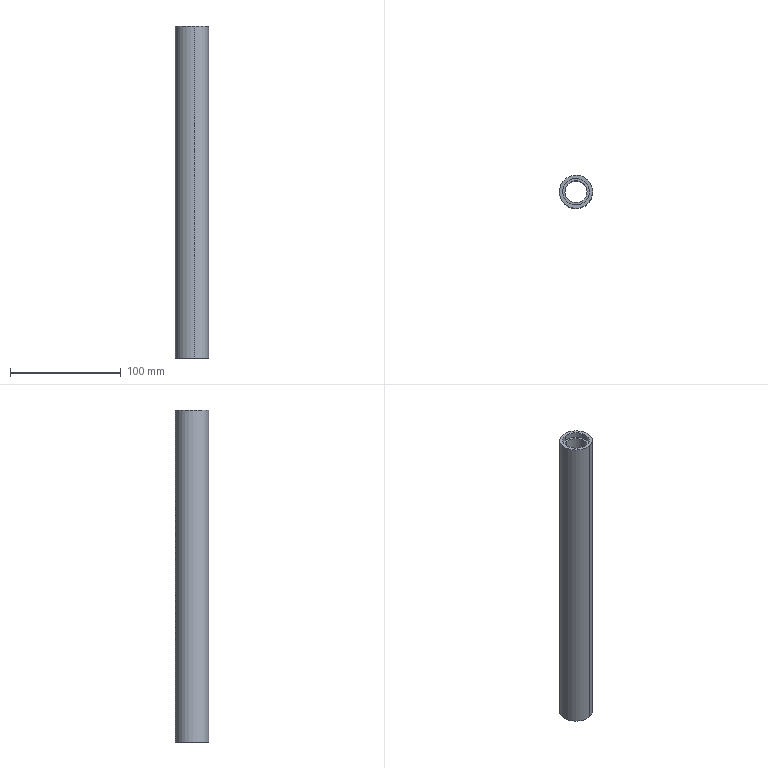Component | SolidWorks | KSD171005A-01-01-25-2 | 1 solid | 12 faces | box 30 x 30 x 300 mm | volume 116427 mm3 | cylinder 8 | plane 4 | commonest cylinder face diameters 24 x4 20 x2 30 x2 | material Aluminum
build123d program:
from build123d import *


with BuildPart() as part:
    # Sketch1 → Revolve1 (revolve)
    with BuildSketch(Plane.XY, mode=Mode.PRIVATE) as revolve1_sk:
        Polygon((0, 12), (0, 15), (300, 15), (300, 12), (295, 12), (295, 10), (5, 10), (5, 12), align=None)
    revolve(revolve1_sk.sketch.rotate(Axis((-43.14, 0, 0), (1, 0, 0)), 90), axis=Axis((-43.14, 0, 0), (1, 0, 0)))


solid = part.part

# Placed as in the assembly
solid = solid.moved(Location((-7.111, -139.27, 933), (0, 90, 0)))
STEP:
#1=CARTESIAN_POINT('',(-0.3647,-5.018,25.118));
#2=VERTEX_POINT('',#1);
#3=CARTESIAN_POINT('',(-0.1952,-5.948,25.118));
#4=VERTEX_POINT('',#3);
#5=CARTESIAN_POINT('',(-0.28,-5.483,25.118));
#6=DIRECTION('',(0.,-0.,-1.));
#7=DIRECTION('',(0.1794,-0.9838,0.));
#8=AXIS2_PLACEMENT_3D('',#5,#6,#7);
#9=CIRCLE('',#8,0.4724);
#10=EDGE_CURVE('',#2,#4,#9,.T.);
#11=ORIENTED_EDGE('',*,*,#10,.F.);
#12=CARTESIAN_POINT('',(-0.3647,-5.018,24.921));
#13=VERTEX_POINT('',#12);
#14=CARTESIAN_POINT('',(-0.3647,-5.018,23.223));
#15=DIRECTION('',(0.,-0.,-1.));
#16=VECTOR('',#15,39.37);
#17=LINE('',#14,#16);
#18=EDGE_CURVE('',#2,#13,#17,.T.);
#19=ORIENTED_EDGE('',*,*,#18,.T.);
#20=CARTESIAN_POINT('',(-0.1952,-5.948,24.921));
#21=VERTEX_POINT('',#20);
#22=CARTESIAN_POINT('',(-0.28,-5.483,24.921));
#23=DIRECTION('',(0.,-0.,-1.));
#24=DIRECTION('',(0.1794,-0.9838,0.));
#25=AXIS2_PLACEMENT_3D('',#22,#23,#24);
#26=CIRCLE('',#25,0.4724);
#27=EDGE_CURVE('',#13,#21,#26,.T.);
#28=ORIENTED_EDGE('',*,*,#27,.T.);
#29=CARTESIAN_POINT('',(-0.1952,-5.948,23.223));
#30=DIRECTION('',(0.,-0.,-1.));
#31=VECTOR('',#30,39.37);
#32=LINE('',#29,#31);
#33=EDGE_CURVE('',#4,#21,#32,.T.);
#34=ORIENTED_EDGE('',*,*,#33,.F.);
#35=EDGE_LOOP('',(#11,#19,#28,#34));
#36=FACE_OUTER_BOUND('',#35,.T.);
#37=CARTESIAN_POINT('',(-0.28,-5.483,23.223));
#38=DIRECTION('',(0.,-0.,-1.));
#39=DIRECTION('',(0.1794,-0.9838,0.));
#40=AXIS2_PLACEMENT_3D('',#37,#38,#39);
#41=CYLINDRICAL_SURFACE('',#40,0.4724);
#42=ADVANCED_FACE('',(#36),#41,.F.);
#43=CARTESIAN_POINT('',(-0.3506,-5.096,36.535));
#44=VERTEX_POINT('',#43);
#45=CARTESIAN_POINT('',(-0.2093,-5.87,36.535));
#46=VERTEX_POINT('',#45);
#47=CARTESIAN_POINT('',(-0.28,-5.483,36.535));
#48=DIRECTION('',(0.,-0.,-1.));
#49=DIRECTION('',(0.1794,-0.9838,0.));
#50=AXIS2_PLACEMENT_3D('',#47,#48,#49);
#51=CIRCLE('',#50,0.3937);
#52=EDGE_CURVE('',#44,#46,#51,.T.);
#53=ORIENTED_EDGE('',*,*,#52,.F.);
#54=CARTESIAN_POINT('',(-0.3506,-5.096,25.118));
#55=VERTEX_POINT('',#54);
#56=CARTESIAN_POINT('',(-0.3506,-5.096,23.223));
#57=DIRECTION('',(0.,-0.,-1.));
#58=VECTOR('',#57,39.37);
#59=LINE('',#56,#58);
#60=EDGE_CURVE('',#44,#55,#59,.T.);
#61=ORIENTED_EDGE('',*,*,#60,.T.);
#62=CARTESIAN_POINT('',(-0.2093,-5.87,25.118));
#63=VERTEX_POINT('',#62);
#64=CARTESIAN_POINT('',(-0.28,-5.483,25.118));
#65=DIRECTION('',(0.,-0.,-1.));
#66=DIRECTION('',(0.1794,-0.9838,0.));
#67=AXIS2_PLACEMENT_3D('',#64,#65,#66);
#68=CIRCLE('',#67,0.3937);
#69=EDGE_CURVE('',#55,#63,#68,.T.);
#70=ORIENTED_EDGE('',*,*,#69,.T.);
#71=CARTESIAN_POINT('',(-0.2093,-5.87,23.223));
#72=DIRECTION('',(0.,-0.,-1.));
#73=VECTOR('',#72,39.37);
#74=LINE('',#71,#73);
#75=EDGE_CURVE('',#46,#63,#74,.T.);
#76=ORIENTED_EDGE('',*,*,#75,.F.);
#77=EDGE_LOOP('',(#53,#61,#70,#76));
#78=FACE_OUTER_BOUND('',#77,.T.);
#79=CARTESIAN_POINT('',(-0.28,-5.483,23.223));
#80=DIRECTION('',(0.,-0.,-1.));
#81=DIRECTION('',(0.1794,-0.9838,0.));
#82=AXIS2_PLACEMENT_3D('',#79,#80,#81);
#83=CYLINDRICAL_SURFACE('',#82,0.3937);
#84=ADVANCED_FACE('',(#78),#83,.F.);
#85=CARTESIAN_POINT('',(-0.3647,-5.018,36.732));
#86=VERTEX_POINT('',#85);
#87=CARTESIAN_POINT('',(-0.1952,-5.948,36.732));
#88=VERTEX_POINT('',#87);
#89=CARTESIAN_POINT('',(-0.28,-5.483,36.732));
#90=DIRECTION('',(0.,-0.,-1.));
#91=DIRECTION('',(0.1794,-0.9838,0.));
#92=AXIS2_PLACEMENT_3D('',#89,#90,#91);
#93=CIRCLE('',#92,0.4724);
#94=EDGE_CURVE('',#86,#88,#93,.T.);
#95=ORIENTED_EDGE('',*,*,#94,.F.);
#96=CARTESIAN_POINT('',(-0.3647,-5.018,36.535));
#97=VERTEX_POINT('',#96);
#98=CARTESIAN_POINT('',(-0.3647,-5.018,23.223));
#99=DIRECTION('',(0.,-0.,-1.));
#100=VECTOR('',#99,39.37);
#101=LINE('',#98,#100);
#102=EDGE_CURVE('',#86,#97,#101,.T.);
#103=ORIENTED_EDGE('',*,*,#102,.T.);
#104=CARTESIAN_POINT('',(-0.1952,-5.948,36.535));
#105=VERTEX_POINT('',#104);
#106=CARTESIAN_POINT('',(-0.28,-5.483,36.535));
#107=DIRECTION('',(0.,-0.,-1.));
#108=DIRECTION('',(0.1794,-0.9838,0.));
#109=AXIS2_PLACEMENT_3D('',#106,#107,#108);
#110=CIRCLE('',#109,0.4724);
#111=EDGE_CURVE('',#97,#105,#110,.T.);
#112=ORIENTED_EDGE('',*,*,#111,.T.);
#113=CARTESIAN_POINT('',(-0.1952,-5.948,23.223));
#114=DIRECTION('',(0.,-0.,-1.));
#115=VECTOR('',#114,39.37);
#116=LINE('',#113,#115);
#117=EDGE_CURVE('',#88,#105,#116,.T.);
#118=ORIENTED_EDGE('',*,*,#117,.F.);
#119=EDGE_LOOP('',(#95,#103,#112,#118));
#120=FACE_OUTER_BOUND('',#119,.T.);
#121=CARTESIAN_POINT('',(-0.28,-5.483,23.223));
#122=DIRECTION('',(0.,-0.,-1.));
#123=DIRECTION('',(0.1794,-0.9838,0.));
#124=AXIS2_PLACEMENT_3D('',#121,#122,#123);
#125=CYLINDRICAL_SURFACE('',#124,0.4724);
#126=ADVANCED_FACE('',(#120),#125,.F.);
#127=CARTESIAN_POINT('',(-0.174,-6.064,36.732));
#128=VERTEX_POINT('',#127);
#129=CARTESIAN_POINT('',(-0.3859,-4.902,36.732));
#130=VERTEX_POINT('',#129);
#131=CARTESIAN_POINT('',(-0.28,-5.483,36.732));
#132=DIRECTION('',(0.,-0.,-1.));
#133=DIRECTION('',(0.1794,-0.9838,0.));
#134=AXIS2_PLACEMENT_3D('',#131,#132,#133);
#135=CIRCLE('',#134,0.5906);
#136=EDGE_CURVE('',#128,#130,#135,.T.);
#137=ORIENTED_EDGE('',*,*,#136,.T.);
#138=CARTESIAN_POINT('',(-0.3859,-4.902,24.921));
#139=VERTEX_POINT('',#138);
#140=CARTESIAN_POINT('',(-0.3859,-4.902,23.223));
#141=DIRECTION('',(0.,-0.,-1.));
#142=VECTOR('',#141,39.37);
#143=LINE('',#140,#142);
#144=EDGE_CURVE('',#130,#139,#143,.T.);
#145=ORIENTED_EDGE('',*,*,#144,.T.);
#146=CARTESIAN_POINT('',(-0.174,-6.064,24.921));
#147=VERTEX_POINT('',#146);
#148=CARTESIAN_POINT('',(-0.28,-5.483,24.921));
#149=DIRECTION('',(0.,-0.,-1.));
#150=DIRECTION('',(0.1794,-0.9838,0.));
#151=AXIS2_PLACEMENT_3D('',#148,#149,#150);
#152=CIRCLE('',#151,0.5906);
#153=EDGE_CURVE('',#147,#139,#152,.T.);
#154=ORIENTED_EDGE('',*,*,#153,.F.);
#155=CARTESIAN_POINT('',(-0.174,-6.064,23.223));
#156=DIRECTION('',(0.,-0.,-1.));
#157=VECTOR('',#156,39.37);
#158=LINE('',#155,#157);
#159=EDGE_CURVE('',#128,#147,#158,.T.);
#160=ORIENTED_EDGE('',*,*,#159,.F.);
#161=EDGE_LOOP('',(#137,#145,#154,#160));
#162=FACE_OUTER_BOUND('',#161,.T.);
#163=CARTESIAN_POINT('',(-0.28,-5.483,23.223));
#164=DIRECTION('',(0.,-0.,-1.));
#165=DIRECTION('',(0.1794,-0.9838,0.));
#166=AXIS2_PLACEMENT_3D('',#163,#164,#165);
#167=CYLINDRICAL_SURFACE('',#166,0.5906);
#168=ADVANCED_FACE('',(#162),#167,.T.);
#169=ORIENTED_EDGE('',*,*,#144,.F.);
#170=CARTESIAN_POINT('',(-0.28,-5.483,36.732));
#171=DIRECTION('',(0.,-0.,-1.));
#172=DIRECTION('',(0.1794,-0.9838,0.));
#173=AXIS2_PLACEMENT_3D('',#170,#171,#172);
#174=CIRCLE('',#173,0.5906);
#175=EDGE_CURVE('',#130,#128,#174,.T.);
#176=ORIENTED_EDGE('',*,*,#175,.T.);
#177=ORIENTED_EDGE('',*,*,#159,.T.);
#178=CARTESIAN_POINT('',(-0.28,-5.483,24.921));
#179=DIRECTION('',(0.,-0.,-1.));
#180=DIRECTION('',(0.1794,-0.9838,0.));
#181=AXIS2_PLACEMENT_3D('',#178,#179,#180);
#182=CIRCLE('',#181,0.5906);
#183=EDGE_CURVE('',#139,#147,#182,.T.);
#184=ORIENTED_EDGE('',*,*,#183,.F.);
#185=EDGE_LOOP('',(#169,#176,#177,#184));
#186=FACE_OUTER_BOUND('',#185,.T.);
#187=CARTESIAN_POINT('',(-0.28,-5.483,23.223));
#188=DIRECTION('',(0.,-0.,-1.));
#189=DIRECTION('',(0.1794,-0.9838,0.));
#190=AXIS2_PLACEMENT_3D('',#187,#188,#189);
#191=CYLINDRICAL_SURFACE('',#190,0.5906);
#192=ADVANCED_FACE('',(#186),#191,.T.);
#193=ORIENTED_EDGE('',*,*,#136,.F.);
#194=ORIENTED_EDGE('',*,*,#175,.F.);
#195=EDGE_LOOP('',(#193,#194));
#196=FACE_OUTER_BOUND('',#195,.T.);
#197=CARTESIAN_POINT('',(-0.28,-5.483,36.732));
#198=DIRECTION('',(0.,-0.,-1.));
#199=DIRECTION('',(0.1794,-0.9838,0.));
#200=AXIS2_PLACEMENT_3D('',#197,#198,#199);
#201=CIRCLE('',#200,0.4724);
#202=EDGE_CURVE('',#88,#86,#201,.T.);
#203=ORIENTED_EDGE('',*,*,#202,.T.);
#204=ORIENTED_EDGE('',*,*,#94,.T.);
#205=EDGE_LOOP('',(#203,#204));
#206=FACE_BOUND('',#205,.T.);
#207=CARTESIAN_POINT('',(-0.8609,-5.589,36.732));
#208=DIRECTION('',(0.,-0.,-1.));
#209=DIRECTION('',(0.1794,-0.9838,0.));
#210=AXIS2_PLACEMENT_3D('',#207,#208,#209);
#211=PLANE('',#210);
#212=ADVANCED_FACE('',(#196,#206),#211,.F.);
#213=ORIENTED_EDGE('',*,*,#102,.F.);
#214=ORIENTED_EDGE('',*,*,#202,.F.);
#215=ORIENTED_EDGE('',*,*,#117,.T.);
#216=CARTESIAN_POINT('',(-0.28,-5.483,36.535));
#217=DIRECTION('',(0.,-0.,-1.));
#218=DIRECTION('',(0.1794,-0.9838,0.));
#219=AXIS2_PLACEMENT_3D('',#216,#217,#218);
#220=CIRCLE('',#219,0.4724);
#221=EDGE_CURVE('',#105,#97,#220,.T.);
#222=ORIENTED_EDGE('',*,*,#221,.T.);
#223=EDGE_LOOP('',(#213,#214,#215,#222));
#224=FACE_OUTER_BOUND('',#223,.T.);
#225=CARTESIAN_POINT('',(-0.28,-5.483,23.223));
#226=DIRECTION('',(0.,-0.,-1.));
#227=DIRECTION('',(0.1794,-0.9838,0.));
#228=AXIS2_PLACEMENT_3D('',#225,#226,#227);
#229=CYLINDRICAL_SURFACE('',#228,0.4724);
#230=ADVANCED_FACE('',(#224),#229,.F.);
#231=ORIENTED_EDGE('',*,*,#221,.F.);
#232=ORIENTED_EDGE('',*,*,#111,.F.);
#233=EDGE_LOOP('',(#231,#232));
#234=FACE_OUTER_BOUND('',#233,.T.);
#235=CARTESIAN_POINT('',(-0.28,-5.483,36.535));
#236=DIRECTION('',(0.,-0.,-1.));
#237=DIRECTION('',(0.1794,-0.9838,0.));
#238=AXIS2_PLACEMENT_3D('',#235,#236,#237);
#239=CIRCLE('',#238,0.3937);
#240=EDGE_CURVE('',#46,#44,#239,.T.);
#241=ORIENTED_EDGE('',*,*,#240,.T.);
#242=ORIENTED_EDGE('',*,*,#52,.T.);
#243=EDGE_LOOP('',(#241,#242));
#244=FACE_BOUND('',#243,.T.);
#245=CARTESIAN_POINT('',(-0.7447,-5.568,36.535));
#246=DIRECTION('',(0.,-0.,-1.));
#247=DIRECTION('',(0.1794,-0.9838,0.));
#248=AXIS2_PLACEMENT_3D('',#245,#246,#247);
#249=PLANE('',#248);
#250=ADVANCED_FACE('',(#234,#244),#249,.F.);
#251=ORIENTED_EDGE('',*,*,#60,.F.);
#252=ORIENTED_EDGE('',*,*,#240,.F.);
#253=ORIENTED_EDGE('',*,*,#75,.T.);
#254=CARTESIAN_POINT('',(-0.28,-5.483,25.118));
#255=DIRECTION('',(0.,-0.,-1.));
#256=DIRECTION('',(0.1794,-0.9838,0.));
#257=AXIS2_PLACEMENT_3D('',#254,#255,#256);
#258=CIRCLE('',#257,0.3937);
#259=EDGE_CURVE('',#63,#55,#258,.T.);
#260=ORIENTED_EDGE('',*,*,#259,.T.);
#261=EDGE_LOOP('',(#251,#252,#253,#260));
#262=FACE_OUTER_BOUND('',#261,.T.);
#263=CARTESIAN_POINT('',(-0.28,-5.483,23.223));
#264=DIRECTION('',(0.,-0.,-1.));
#265=DIRECTION('',(0.1794,-0.9838,0.));
#266=AXIS2_PLACEMENT_3D('',#263,#264,#265);
#267=CYLINDRICAL_SURFACE('',#266,0.3937);
#268=ADVANCED_FACE('',(#262),#267,.F.);
#269=ORIENTED_EDGE('',*,*,#259,.F.);
#270=ORIENTED_EDGE('',*,*,#69,.F.);
#271=EDGE_LOOP('',(#269,#270));
#272=FACE_BOUND('',#271,.T.);
#273=CARTESIAN_POINT('',(-0.28,-5.483,25.118));
#274=DIRECTION('',(0.,-0.,-1.));
#275=DIRECTION('',(0.1794,-0.9838,0.));
#276=AXIS2_PLACEMENT_3D('',#273,#274,#275);
#277=CIRCLE('',#276,0.4724);
#278=EDGE_CURVE('',#4,#2,#277,.T.);
#279=ORIENTED_EDGE('',*,*,#278,.T.);
#280=ORIENTED_EDGE('',*,*,#10,.T.);
#281=EDGE_LOOP('',(#279,#280));
#282=FACE_OUTER_BOUND('',#281,.T.);
#283=CARTESIAN_POINT('',(-0.6673,-5.554,25.118));
#284=DIRECTION('',(-0.,0.,1.));
#285=DIRECTION('',(-0.1794,0.9838,-0.));
#286=AXIS2_PLACEMENT_3D('',#283,#284,#285);
#287=PLANE('',#286);
#288=ADVANCED_FACE('',(#272,#282),#287,.F.);
#289=ORIENTED_EDGE('',*,*,#18,.F.);
#290=ORIENTED_EDGE('',*,*,#278,.F.);
#291=ORIENTED_EDGE('',*,*,#33,.T.);
#292=CARTESIAN_POINT('',(-0.28,-5.483,24.921));
#293=DIRECTION('',(0.,-0.,-1.));
#294=DIRECTION('',(0.1794,-0.9838,0.));
#295=AXIS2_PLACEMENT_3D('',#292,#293,#294);
#296=CIRCLE('',#295,0.4724);
#297=EDGE_CURVE('',#21,#13,#296,.T.);
#298=ORIENTED_EDGE('',*,*,#297,.T.);
#299=EDGE_LOOP('',(#289,#290,#291,#298));
#300=FACE_OUTER_BOUND('',#299,.T.);
#301=CARTESIAN_POINT('',(-0.28,-5.483,23.223));
#302=DIRECTION('',(0.,-0.,-1.));
#303=DIRECTION('',(0.1794,-0.9838,0.));
#304=AXIS2_PLACEMENT_3D('',#301,#302,#303);
#305=CYLINDRICAL_SURFACE('',#304,0.4724);
#306=ADVANCED_FACE('',(#300),#305,.F.);
#307=ORIENTED_EDGE('',*,*,#297,.F.);
#308=ORIENTED_EDGE('',*,*,#27,.F.);
#309=EDGE_LOOP('',(#307,#308));
#310=FACE_BOUND('',#309,.T.);
#311=ORIENTED_EDGE('',*,*,#153,.T.);
#312=ORIENTED_EDGE('',*,*,#183,.T.);
#313=EDGE_LOOP('',(#311,#312));
#314=FACE_OUTER_BOUND('',#313,.T.);
#315=CARTESIAN_POINT('',(-0.7447,-5.568,24.921));
#316=DIRECTION('',(-0.,0.,1.));
#317=DIRECTION('',(-0.1794,0.9838,-0.));
#318=AXIS2_PLACEMENT_3D('',#315,#316,#317);
#319=PLANE('',#318);
#320=ADVANCED_FACE('',(#310,#314),#319,.F.);
#321=CLOSED_SHELL('',(#42,#84,#126,#168,#192,#212,#230,#250,#268,#288,#306,#320));
#322=MANIFOLD_SOLID_BREP('',#321);
#323=CARTESIAN_POINT('',(0.,0.,0.));
#324=DIRECTION('',(0.,0.,1.));
#325=DIRECTION('',(1.,0.,0.));
#326=AXIS2_PLACEMENT_3D('',#323,#324,#325);
#327=(LENGTH_UNIT()NAMED_UNIT(*)SI_UNIT($,.METRE.));
#328=LENGTH_MEASURE_WITH_UNIT(LENGTH_MEASURE(0.0254),#327);
#329=DIMENSIONAL_EXPONENTS(1.,0.,0.,0.,0.,0.,0.);
#330=(CONVERSION_BASED_UNIT('',#328)LENGTH_UNIT()NAMED_UNIT(#329));
#331=UNCERTAINTY_MEASURE_WITH_UNIT(LENGTH_MEASURE(0.00001),#330,'','');
#332=(NAMED_UNIT(*)PLANE_ANGLE_UNIT()SI_UNIT($,.RADIAN.));
#333=(NAMED_UNIT(*)SI_UNIT($,.STERADIAN.)SOLID_ANGLE_UNIT());
#334=(GEOMETRIC_REPRESENTATION_CONTEXT(3)GLOBAL_UNCERTAINTY_ASSIGNED_CONTEXT((#331))GLOBAL_UNIT_ASSIGNED_CONTEXT((#330,#332,#333))REPRESENTATION_CONTEXT('',''));
#335=ADVANCED_BREP_SHAPE_REPRESENTATION('',(#322,#326),#334);
#336=COLOUR_RGB('',0.7922,0.8196,0.9333);
#337=FILL_AREA_STYLE_COLOUR('',#336);
#338=FILL_AREA_STYLE('',(#337));
#339=SURFACE_STYLE_FILL_AREA(#338);
#340=SURFACE_SIDE_STYLE('',(#339));
#341=SURFACE_STYLE_USAGE(.BOTH.,#340);
#342=PRESENTATION_STYLE_ASSIGNMENT((#341));
#343=STYLED_ITEM('',(#342),#322);
#344=PRESENTATION_LAYER_ASSIGNMENT('','',(#343));
#345=(LENGTH_UNIT()NAMED_UNIT(*)SI_UNIT($,.METRE.));
#346=LENGTH_MEASURE_WITH_UNIT(LENGTH_MEASURE(0.0254),#345);
#347=DIMENSIONAL_EXPONENTS(1.,0.,0.,0.,0.,0.,0.);
#348=(CONVERSION_BASED_UNIT('',#346)LENGTH_UNIT()NAMED_UNIT(#347));
#349=UNCERTAINTY_MEASURE_WITH_UNIT(LENGTH_MEASURE(0.00001),#348,'','');
#350=(NAMED_UNIT(*)PLANE_ANGLE_UNIT()SI_UNIT($,.RADIAN.));
#351=(NAMED_UNIT(*)SI_UNIT($,.STERADIAN.)SOLID_ANGLE_UNIT());
#352=(GEOMETRIC_REPRESENTATION_CONTEXT(3)GLOBAL_UNCERTAINTY_ASSIGNED_CONTEXT((#349))GLOBAL_UNIT_ASSIGNED_CONTEXT((#348,#350,#351))REPRESENTATION_CONTEXT('',''));
#353=MECHANICAL_DESIGN_GEOMETRIC_PRESENTATION_REPRESENTATION('',(#343),#352);